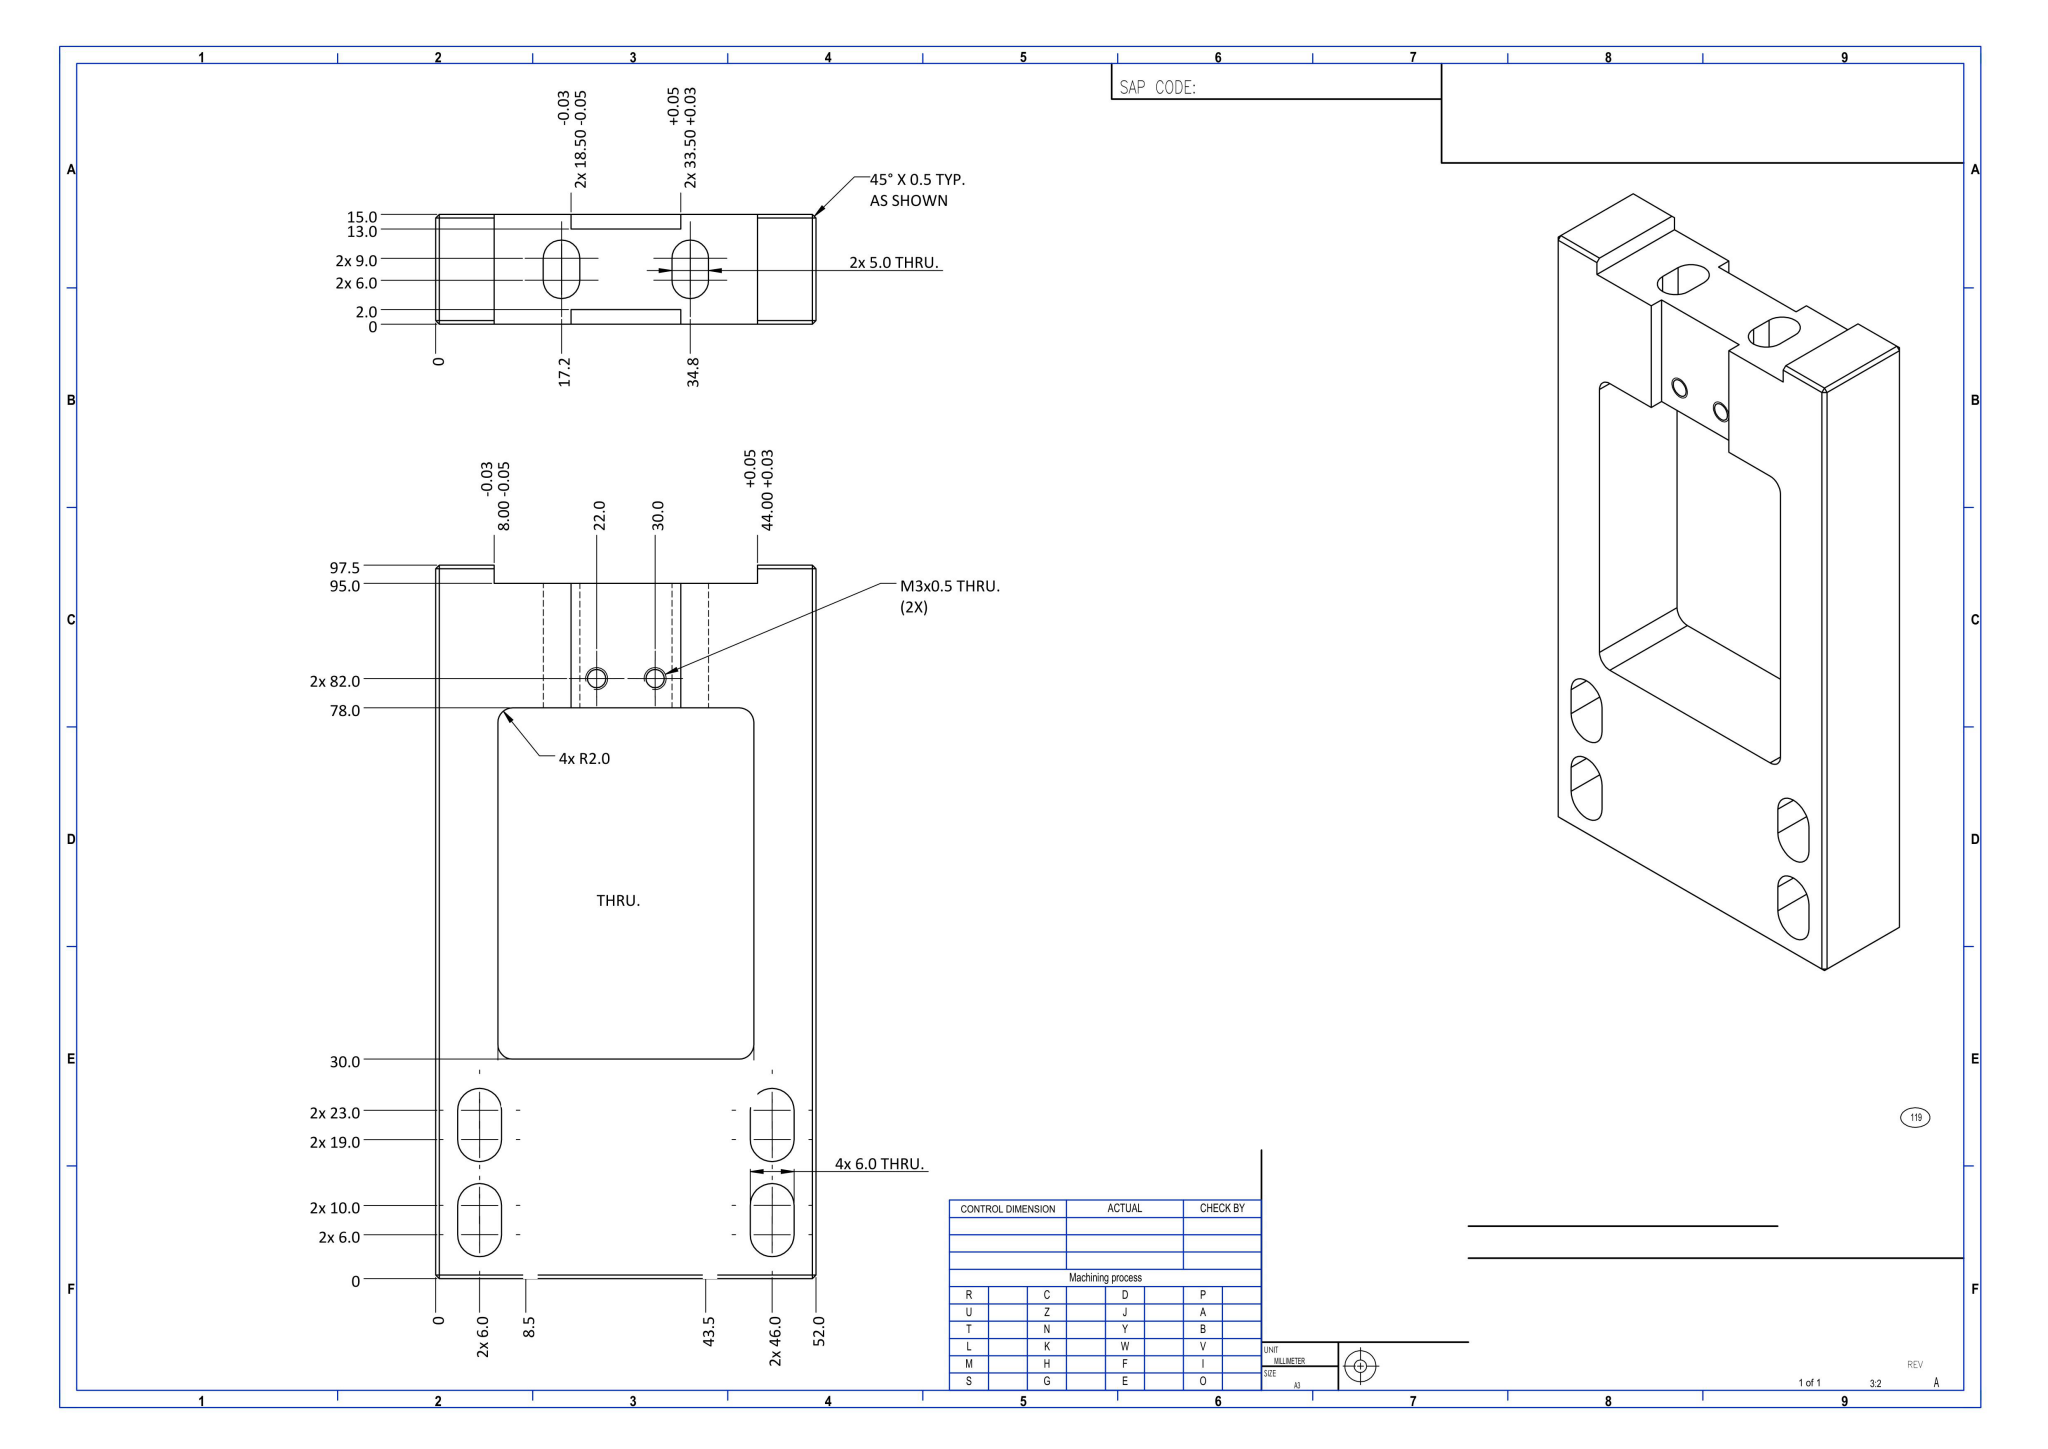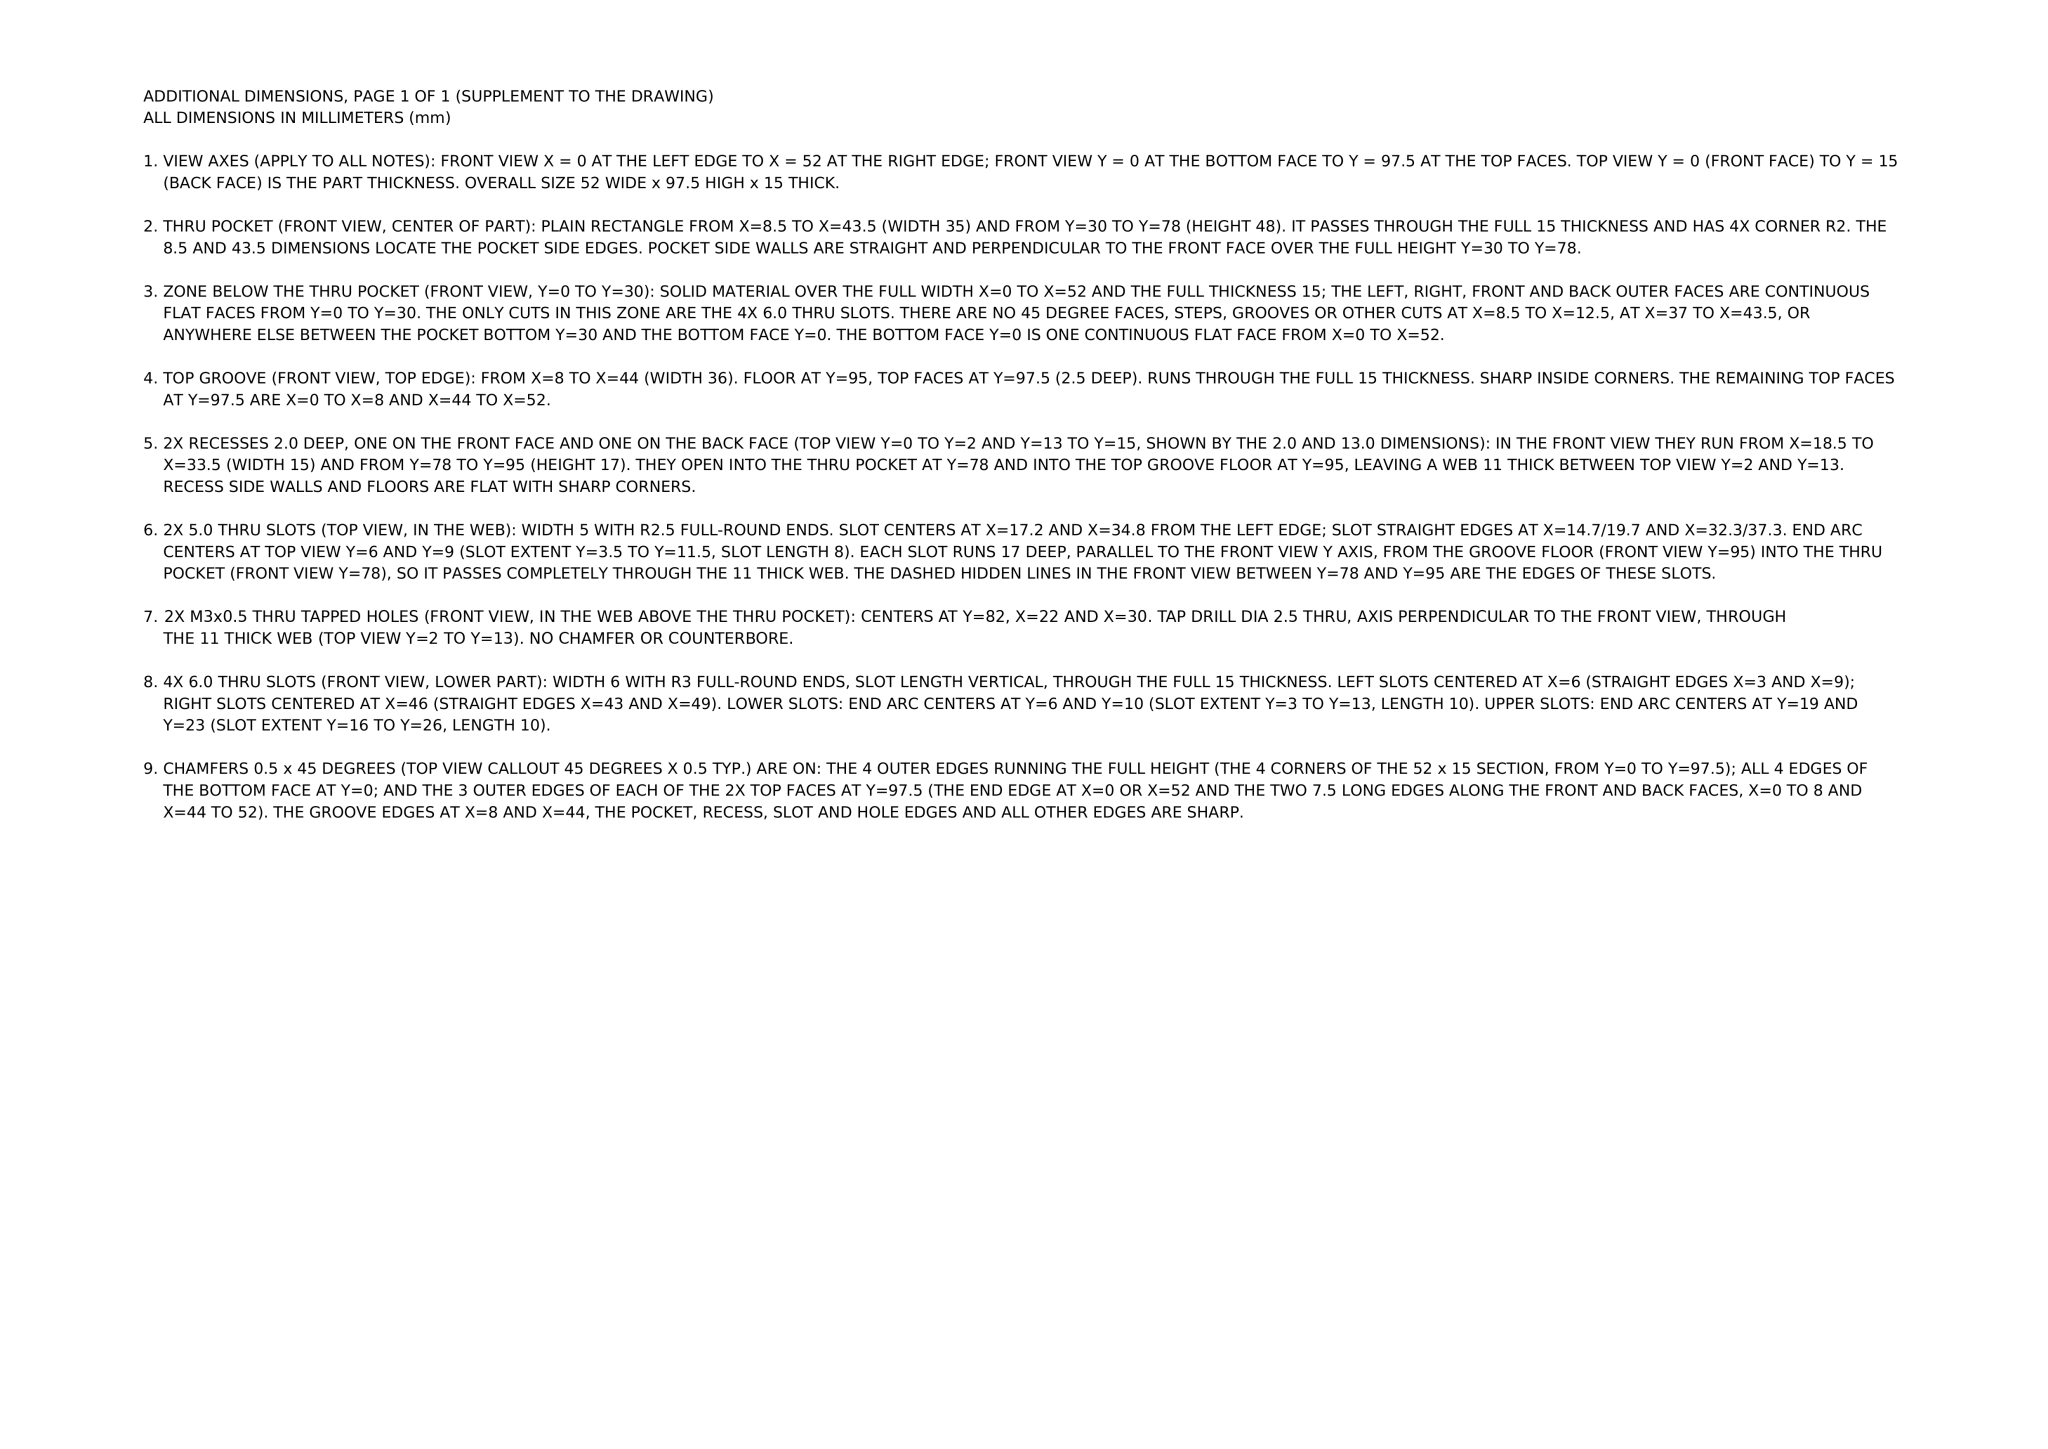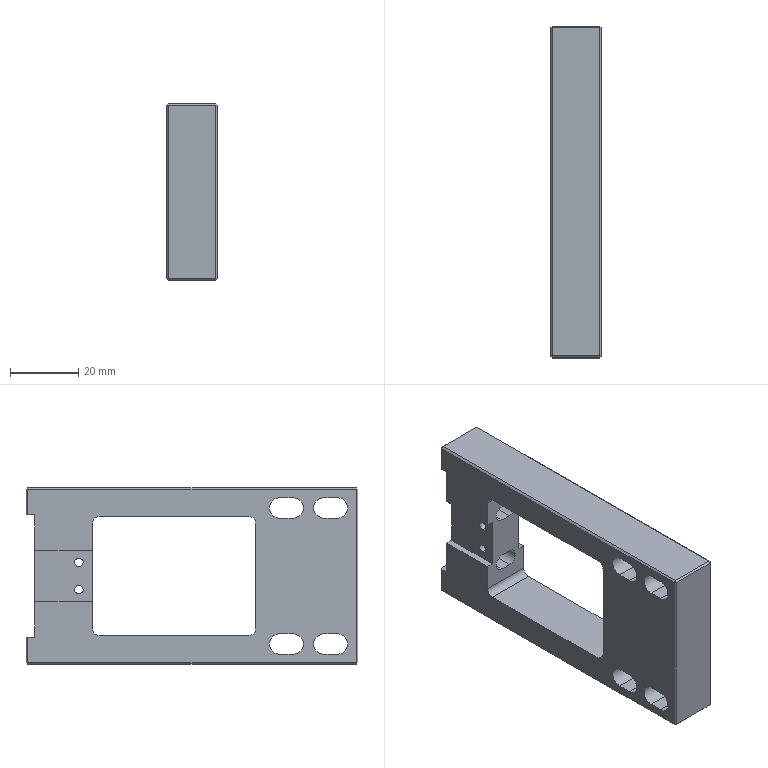Part | NX | mm | 1 solid | 74 faces | box 15 x 97.5 x 52 mm | volume 44037 mm3 | plane 54 | cylinder 20 | commonest cylinder face diameters 6 x8 2.5 x4 5 x4 4 x4